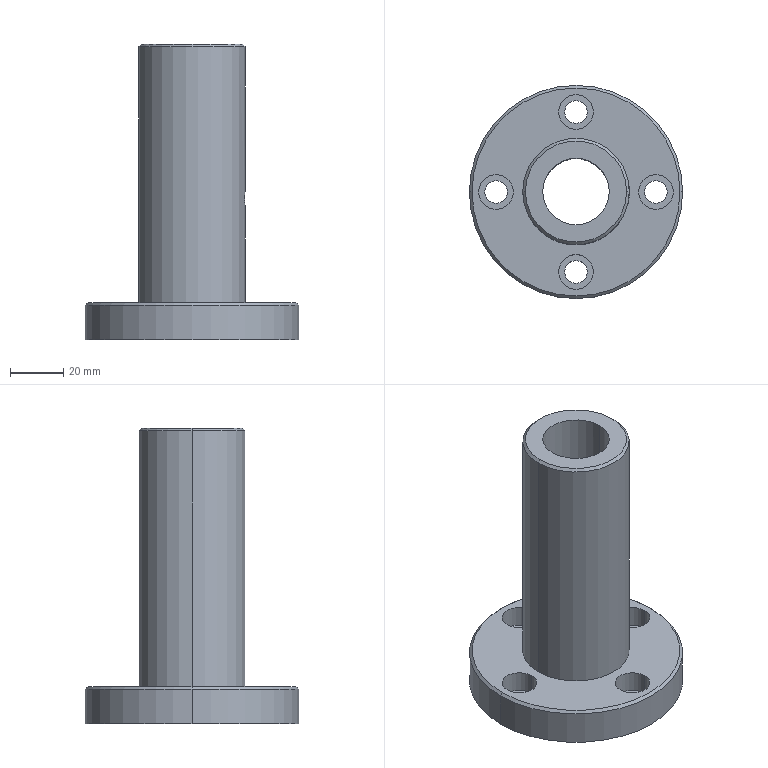Component | SolidWorks | DirectPressureVerticalSeal-1_FlangeSeat-1 | 1 solid | 35 faces | box 80 x 80 x 111 mm | volume 131709 mm3 | cylinder 24 | plane 7 | cone 4 | commonest cylinder face diameters 13 x8 8.5 x8 6.8 x2 25 x2 40 x2 80 x2
build123d program:
from build123d import *

# Parameters (mm, degrees)
SKETCH1_W                                            = 14
SKETCH1_H                                            = 40
SKETCH2_R                                            = 20
BOSS_EXTRUDE1_DEPTH                                  = 97
F_25_0_25_DIAMETER_HOLE1_D                           = 25
F_6_8_6_8_DIAMETER_HOLE1_REACH                       = 94.542
F_6_8_6_8_DIAMETER_HOLE1_BORE_R                      = 3.4
CYLINDRICAL_COUNTERSUNK_HOLE_1_FOR_M8_HE_D           = 8.5
CYLINDRICAL_COUNTERSUNK_HOLE_1_FOR_M8_HE_CBORE_D     = 13
CYLINDRICAL_COUNTERSUNK_HOLE_1_FOR_M8_HE_CBORE_DEPTH = 8
CHAMFER1_SIZE                                        = 1


with BuildPart() as part:
    # Sketch1 → Revolve1 (revolve)
    with BuildSketch(Plane(origin=(0, 0, 0), x_dir=(-1, 0, 0), z_dir=(0, 0, -1)), mode=Mode.PRIVATE) as revolve1_sk:
        with Locations((7, 20)):
            Rectangle(SKETCH1_W, SKETCH1_H)
    revolve(revolve1_sk.sketch.rotate(Axis((0, 0, 0), (-1, 0, 0)), 270), axis=Axis((0, 0, 0), (-1, 0, 0)))

    # Sketch2 → Boss-Extrude1 (add)
    with BuildSketch(Plane.ZY.offset(14)):
        with Locations(Location((0, 0, 0), (0, 0, 180))):
            Circle(SKETCH2_R)
    extrude(amount=BOSS_EXTRUDE1_DEPTH)

    # 25.0 _25_ Diameter Hole1 (through all)
    with Locations(Plane(origin=(0, 0, 0), x_dir=(0, 0, -1), z_dir=(1, 0, 0))):
        with Locations((0, 0)):
            Hole(F_25_0_25_DIAMETER_HOLE1_D / 2)

    # 6.8 _6.8_ Diameter Hole1 bore (on position points) → 6.8 _6.8_ Diameter Hole1 (cut, up to next)
    with BuildSketch(Plane(origin=(-53, 0, 20), x_dir=(1, 0, 0), z_dir=(0, 0, 1)), mode=Mode.PRIVATE) as f_6_8_6_8_diameter_hole1_sk1:
        Circle(F_6_8_6_8_DIAMETER_HOLE1_BORE_R)
    f_6_8_6_8_diameter_hole1_tool1 = extrude(f_6_8_6_8_diameter_hole1_sk1.sketch, amount=-F_6_8_6_8_DIAMETER_HOLE1_REACH, mode=Mode.PRIVATE) & part.part
    add(f_6_8_6_8_diameter_hole1_tool1.solids().sort_by_distance((-53, 0, 20))[0], mode=Mode.SUBTRACT)

    # Cylindrical Countersunk Hole 1 for M8 He (through all)
    with Locations(Plane.ZY.offset(14)):
        with Locations((0, 30), (30, 0), (-30, 0), (0, -30)):
            CounterBoreHole(CYLINDRICAL_COUNTERSUNK_HOLE_1_FOR_M8_HE_D / 2, CYLINDRICAL_COUNTERSUNK_HOLE_1_FOR_M8_HE_CBORE_D / 2, CYLINDRICAL_COUNTERSUNK_HOLE_1_FOR_M8_HE_CBORE_DEPTH)

    # Chamfer1
    chamfer1_edges = [part.edges().sort_by_distance(p)[0] for p in [
        (-111, 0, 20),
        (-14, 0, -40),
    ]]
    chamfer(chamfer1_edges, length=CHAMFER1_SIZE)


solid = part.part

# Placed as in the assembly
solid = solid.moved(Location((-98.746, 246.873, -16.5), (0, 90, 0)))